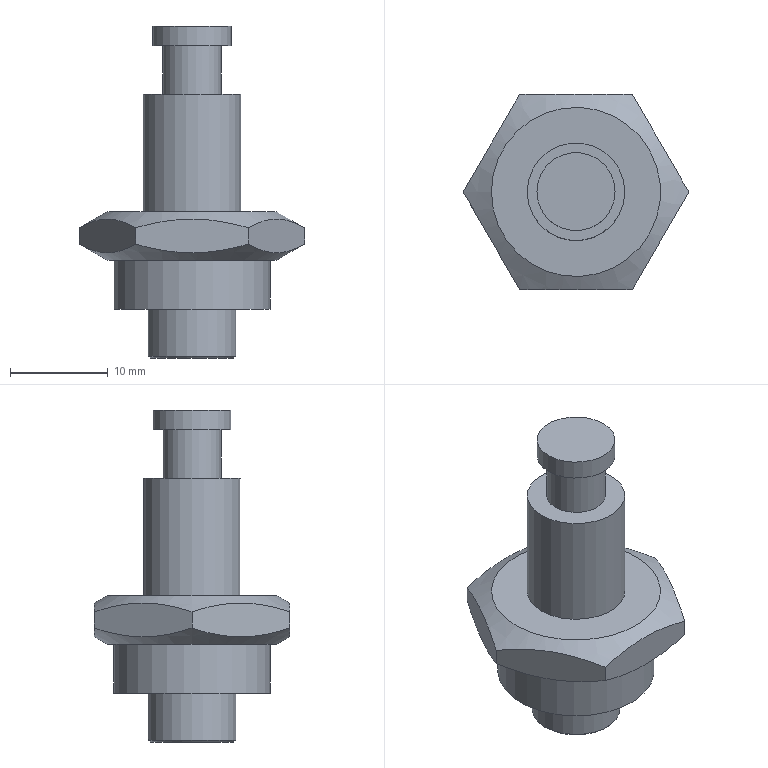Component | NX | SPARK_PLUG | 1 solid | 21 faces | volume 4109 mm3 | plane 13 | cylinder 5 | cone 3 | commonest cylinder face diameters 9 x1 16 x1 10 x1 6 x1 8 x1